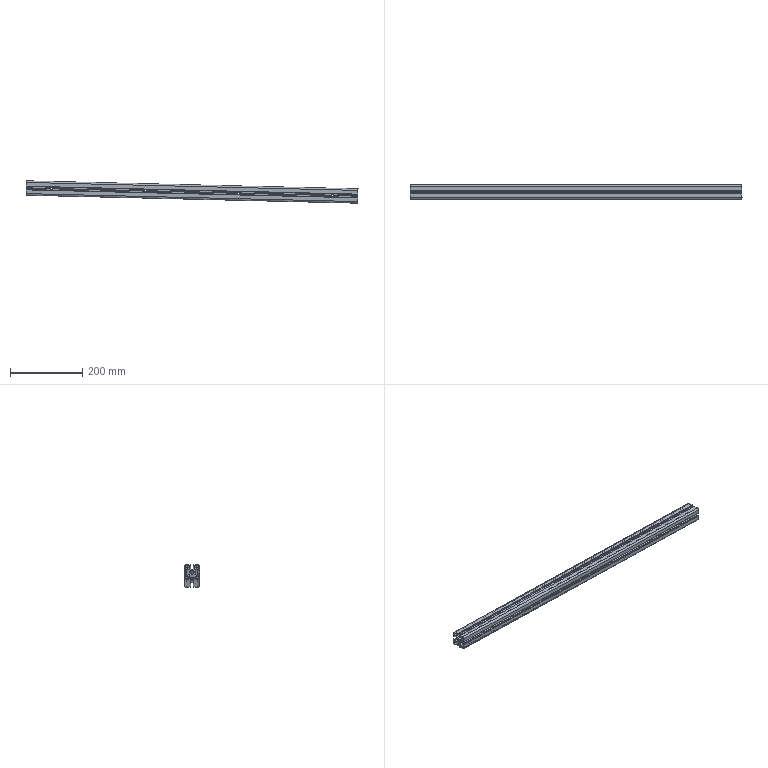Component | SolidWorks | 2012MB0201-1_AUpperRackFrameModule-1_A3006-0-1 | 1 solid | 307 faces | box 920.69 x 40 x 62 mm | volume 547978 mm3 | plane 211 | cylinder 96 | commonest cylinder face diameters 6.6 x32 6.8 x15 2 x12 19 x10 1 x8 11 x8 9 x4 5 x4
build123d program:
from build123d import *

# Parameters (mm, degrees)
BOSS_EXTRUDE1_DEPTH                                  = 920
SKETCH2_R                                            = 9.5
CUT_EXTRUDE1_DEPTH                                   = 18
M6_HEX_SOCKET_HEAD_CAP_SCREW_COUNTERBORE_D           = 6.6
M6_HEX_SOCKET_HEAD_CAP_SCREW_COUNTERBORE_CBORE_D     = 11
M6_HEX_SOCKET_HEAD_CAP_SCREW_COUNTERBORE_CBORE_DEPTH = 6.8


with BuildPart() as part:
    # Sketch1 → Boss-Extrude1 (new body)
    with BuildSketch(Plane.XY):
        with BuildLine():
            Line((-19, -4.1), (-19, -5.1))
            Line((-19, -5.1), (-20, -5.1))
            Line((-20, -5.1), (-20, -15.5))
            ThreePointArc((-20, -15.5), (-18.681, -18.682), (-15.499, -20))
            Line((-15.499, -20), (-5.099, -20))
            Line((-5.099, -20), (-5.099, -19))
            Line((-5.099, -19), (-4.099, -19))
            Line((-4.099, -19), (-4.099, -15.5))
            Line((-4.099, -15.5), (-6.599, -15.5))
            Line((-6.599, -15.5), (-6.599, -16.5))
            ThreePointArc((-6.599, -16.5), (-6.892, -17.207), (-7.599, -17.5))
            Line((-7.599, -17.5), (-9.8, -17.5))
            ThreePointArc((-9.8, -17.5), (-10.153, -17.354), (-10.3, -17))
            Line((-10.3, -17), (-10.3, -11.997))
            Line((-10.3, -11.997), (-5.902, -7.6))
            Line((-5.902, -7.6), (-0.5195, -7.6))
            Line((-0.5195, -7.6), (0.0005, -7.3))
            Line((0.0005, -7.3), (0.5195, -7.6))
            Line((0.5195, -7.6), (5.904, -7.6))
            Line((5.904, -7.6), (10.3, -11.997))
            Line((10.3, -11.997), (10.3, -17))
            ThreePointArc((10.3, -17), (10.154, -17.354), (9.8, -17.5))
            Line((9.8, -17.5), (7.601, -17.5))
            ThreePointArc((7.601, -17.5), (6.893, -17.207), (6.601, -16.5))
            Line((6.601, -16.5), (6.601, -15.5))
            Line((6.601, -15.5), (4.101, -15.5))
            Line((4.101, -15.5), (4.101, -19))
            Line((4.101, -19), (5.101, -19))
            Line((5.101, -19), (5.101, -20))
            Line((5.101, -20), (15.501, -20))
            ThreePointArc((15.501, -20), (18.682, -18.682), (20, -15.5))
            Line((20, -15.5), (20, -5.1))
            Line((20, -5.1), (19, -5.1))
            Line((19, -5.1), (19, -4.1))
            Line((19, -4.1), (15.501, -4.1))
            Line((15.501, -4.1), (15.501, -6.6))
            Line((15.501, -6.6), (16.5, -6.6))
            ThreePointArc((16.5, -6.6), (17.208, -6.893), (17.5, -7.6))
            Line((17.5, -7.6), (17.5, -9.8))
            ThreePointArc((17.5, -9.8), (17.354, -10.154), (17, -10.3))
            Line((17, -10.3), (11.998, -10.3))
            Line((11.998, -10.3), (7.601, -5.903))
            Line((7.601, -5.903), (7.601, -0.5203))
            Line((7.601, -0.5203), (7.301, -0.0003417))
            Line((7.301, -0.0003417), (7.601, 0.5197))
            Line((7.601, 0.5197), (7.601, 5.903))
            Line((7.601, 5.903), (11.998, 10.3))
            Line((11.998, 10.3), (17, 10.3))
            ThreePointArc((17, 10.3), (17.354, 10.153), (17.5, 9.8))
            Line((17.5, 9.8), (17.5, 7.6))
            ThreePointArc((17.5, 7.6), (17.208, 6.893), (16.5, 6.6))
            Line((16.5, 6.6), (15.501, 6.6))
            Line((15.501, 6.6), (15.501, 4.1))
            Line((15.501, 4.1), (19, 4.1))
            Line((19, 4.1), (19, 5.1))
            Line((19, 5.1), (20, 5.1))
            Line((20, 5.1), (20, 15.5))
            ThreePointArc((20, 15.5), (18.682, 18.682), (15.501, 20))
            Line((15.501, 20), (5.101, 20))
            Line((5.101, 20), (5.101, 19))
            Line((5.101, 19), (4.101, 19))
            Line((4.101, 19), (4.101, 15.5))
            Line((4.101, 15.5), (6.601, 15.5))
            ThreePointArc((6.601, 15.5), (6.393, 16), (6.601, 16.5))
            ThreePointArc((6.601, 16.5), (6.893, 17.207), (7.601, 17.5))
            Line((7.601, 17.5), (9.8, 17.5))
            ThreePointArc((9.8, 17.5), (10.154, 17.353), (10.3, 17))
            Line((10.3, 17), (10.3, 11.997))
            Line((10.3, 11.997), (5.904, 7.6))
            Line((5.904, 7.6), (0.5195, 7.6))
            Line((0.5195, 7.6), (0.0005, 7.3))
            Line((0.0005, 7.3), (-0.5195, 7.6))
            Line((-0.5195, 7.6), (-5.902, 7.6))
            Line((-5.902, 7.6), (-10.3, 11.997))
            Line((-10.3, 11.997), (-10.3, 17))
            ThreePointArc((-10.3, 17), (-10.153, 17.353), (-9.8, 17.5))
            Line((-9.8, 17.5), (-7.599, 17.5))
            ThreePointArc((-7.599, 17.5), (-6.892, 17.207), (-6.599, 16.5))
            Line((-6.599, 16.5), (-6.599, 15.5))
            Line((-6.599, 15.5), (-4.099, 15.5))
            Line((-4.099, 15.5), (-4.099, 19))
            Line((-4.099, 19), (-5.099, 19))
            Line((-5.099, 19), (-5.099, 20))
            Line((-5.099, 20), (-15.499, 20))
            ThreePointArc((-15.499, 20), (-18.681, 18.682), (-20, 15.5))
            Line((-20, 15.5), (-20, 5.1))
            Line((-20, 5.1), (-19, 5.1))
            Line((-19, 5.1), (-19, 4.1))
            Line((-19, 4.1), (-15.499, 4.1))
            Line((-15.499, 4.1), (-15.499, 6.6))
            Line((-15.499, 6.6), (-16.5, 6.6))
            ThreePointArc((-16.5, 6.6), (-17.207, 6.893), (-17.5, 7.6))
            Line((-17.5, 7.6), (-17.5, 9.8))
            ThreePointArc((-17.5, 9.8), (-17.353, 10.153), (-17, 10.3))
            Line((-17, 10.3), (-11.996, 10.3))
            Line((-11.996, 10.3), (-7.599, 5.903))
            Line((-7.599, 5.903), (-7.599, 0.5197))
            Line((-7.599, 0.5197), (-7.3, -0.0003417))
            Line((-7.3, -0.0003417), (-7.599, -0.5203))
            Line((-7.599, -0.5203), (-7.599, -5.903))
            Line((-7.599, -5.903), (-11.996, -10.3))
            Line((-11.996, -10.3), (-17, -10.3))
            ThreePointArc((-17, -10.3), (-17.353, -10.154), (-17.5, -9.8))
            Line((-17.5, -9.8), (-17.5, -7.6))
            ThreePointArc((-17.5, -7.6), (-17.207, -6.893), (-16.5, -6.6))
            Line((-16.5, -6.6), (-15.499, -6.6))
            Line((-15.499, -6.6), (-15.499, -4.1))
            Line((-15.499, -4.1), (-19, -4.1))
        make_face()
        with BuildLine():
            Line((15.501, -18), (11.8, -18))
            Line((11.8, -18), (11.8, -11.8))
            Line((11.8, -11.8), (18, -11.8))
            Line((18, -11.8), (18, -15.5))
            ThreePointArc((18, -15.5), (17.268, -17.268), (15.501, -18))
        make_face(mode=Mode.SUBTRACT)
        with BuildLine():
            Line((18, 11.8), (11.8, 11.8))
            Line((11.8, 11.8), (11.8, 18))
            Line((11.8, 18), (15.501, 18))
            ThreePointArc((15.501, 18), (17.268, 17.267), (18, 15.5))
            Line((18, 15.5), (18, 11.8))
        make_face(mode=Mode.SUBTRACT)
        with BuildLine():
            Line((-1.815, -2.875), (-3.004, -4.066))
            Line((-3.004, -4.066), (-4.066, -3.005))
            Line((-4.066, -3.005), (-2.874, -1.815))
            ThreePointArc((-2.874, -1.815), (-3.399, -0.0003417), (-2.874, 1.815))
            Line((-2.874, 1.815), (-4.064, 3.006))
            Line((-4.064, 3.006), (-3.004, 4.066))
            Line((-3.004, 4.066), (-1.815, 2.875))
            ThreePointArc((-1.815, 2.875), (0, 3.399), (1.815, 2.875))
            Line((1.815, 2.875), (3.006, 4.066))
            Line((3.006, 4.066), (4.067, 3.005))
            Line((4.067, 3.005), (2.876, 1.815))
            ThreePointArc((2.876, 1.815), (3.4, -0.0003417), (2.876, -1.815))
            Line((2.876, -1.815), (4.067, -3.005))
            Line((4.067, -3.005), (3.006, -4.066))
            Line((3.006, -4.066), (1.815, -2.875))
            ThreePointArc((1.815, -2.875), (0, -3.4), (-1.815, -2.875))
        make_face(mode=Mode.SUBTRACT)
        with BuildLine():
            Line((-18, -15.5), (-18, -11.8))
            Line((-18, -11.8), (-11.8, -11.8))
            Line((-11.8, -11.8), (-11.8, -18))
            Line((-11.8, -18), (-15.499, -18))
            ThreePointArc((-15.499, -18), (-17.267, -17.268), (-18, -15.5))
        make_face(mode=Mode.SUBTRACT)
        with BuildLine():
            Line((-11.8, 18), (-11.8, 11.8))
            Line((-11.8, 11.8), (-18, 11.8))
            Line((-18, 11.8), (-18, 15.5))
            ThreePointArc((-18, 15.5), (-17.267, 17.267), (-15.499, 18))
            Line((-15.499, 18), (-11.8, 18))
        make_face(mode=Mode.SUBTRACT)
    extrude(amount=-BOSS_EXTRUDE1_DEPTH)

    # Sketch2 → Cut-Extrude1 (cut)
    with BuildSketch(Plane(origin=(0, 20, 0), x_dir=(1, 0, 0), z_dir=(0, 1, 0))):
        with Locations(Location((0, 19, 0), (0, 0, 216.875))):
            Circle(SKETCH2_R)
        with Locations(Location((0, 901, 0), (0, 0, 216.875))):
            Circle(SKETCH2_R)
    extrude(amount=-CUT_EXTRUDE1_DEPTH, mode=Mode.SUBTRACT)

    # M6 Hex Socket Head Cap Screw Counterbore (through all)
    with Locations(Plane(origin=(0.0005, 20, -70), x_dir=(1, 0, 0), z_dir=(0, 1, 0))):
        with Locations((0, 0), (0, 780), (0, 520), (0, 260)):
            CounterBoreHole(M6_HEX_SOCKET_HEAD_CAP_SCREW_COUNTERBORE_D / 2, M6_HEX_SOCKET_HEAD_CAP_SCREW_COUNTERBORE_CBORE_D / 2, M6_HEX_SOCKET_HEAD_CAP_SCREW_COUNTERBORE_CBORE_DEPTH)


solid = part.part

# Placed as in the assembly
solid = solid.moved(Location((-1764.93, -61.149, -1140.065), (0, -88.629, 0)))